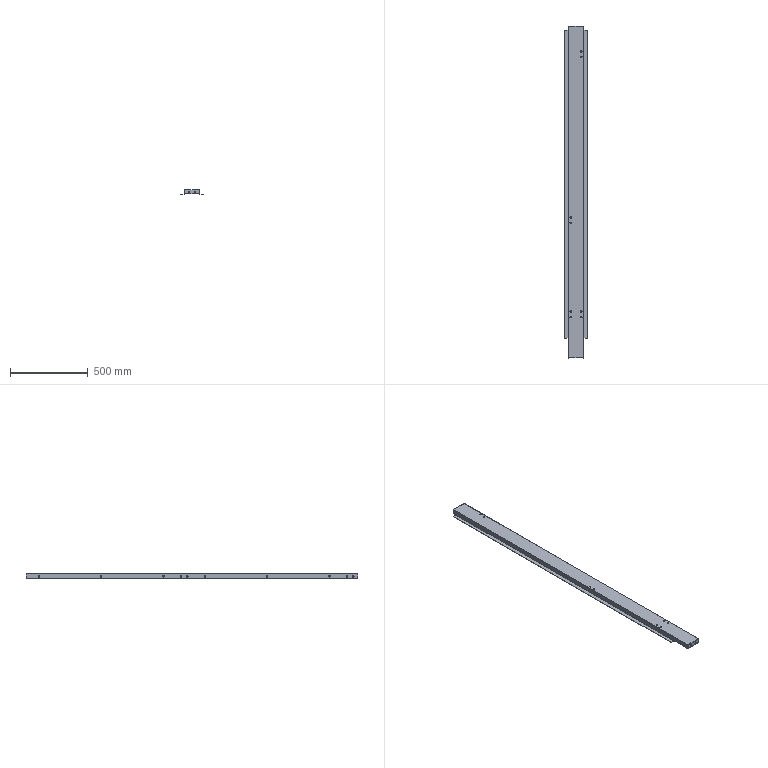Component | SolidWorks | 17FrontMiddleColumn-2 | 1 solid | 126 faces | volume 867789 mm3 | cylinder 76 | plane 50 | commonest cylinder face diameters 10 x64 6 x6 2 x6